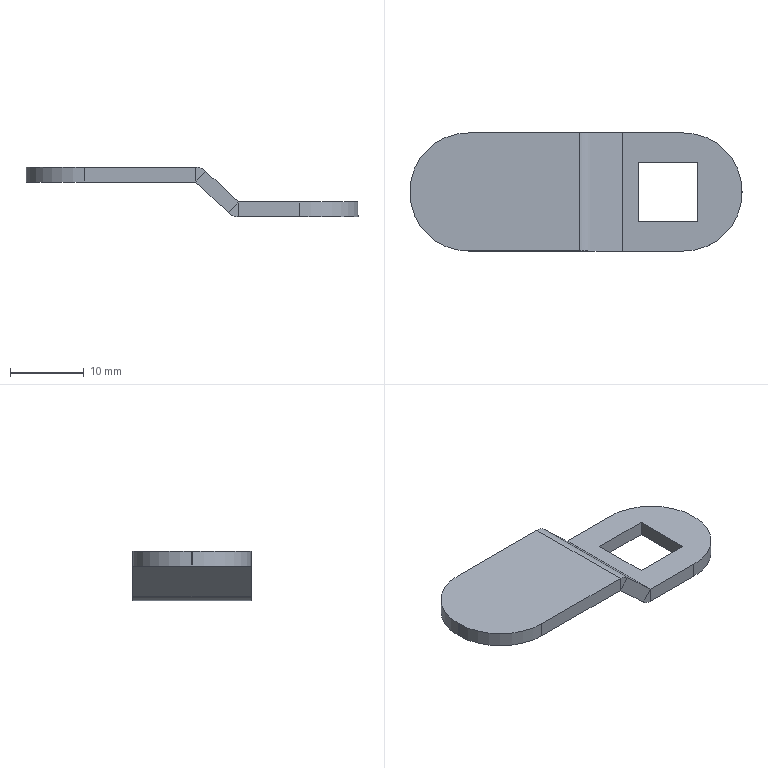Component | SolidWorks | LeftDoorPanelAssembly-1_LockPlate-1 | 1 solid | 30 faces | box 45 x 16 x 6.7 mm | volume 1262 mm3 | plane 22 | cylinder 8 | commonest cylinder face diameters 15.8 x4 0.08 x2 4.08 x2
STEP:
#1=COLOUR_RGB('',0.7922,0.8196,0.9333);
#2=FILL_AREA_STYLE_COLOUR('',#1);
#3=FILL_AREA_STYLE('',(#2));
#4=SURFACE_STYLE_FILL_AREA(#3);
#5=SURFACE_SIDE_STYLE('',(#4));
#6=SURFACE_STYLE_USAGE(.BOTH.,#5);
#7=PRESENTATION_STYLE_ASSIGNMENT((#6));
#8=CARTESIAN_POINT('',(-0.2747,0.2182,-2.108));
#9=VERTEX_POINT('',#8);
#10=CARTESIAN_POINT('',(-0.2208,0.2182,-2.051));
#11=VERTEX_POINT('',#10);
#12=CARTESIAN_POINT('',(-0.2747,0.2182,-2.108));
#13=DIRECTION('',(0.6849,0.,0.7286));
#14=VECTOR('',#13,39.37);
#15=LINE('',#12,#14);
#16=EDGE_CURVE('',#9,#11,#15,.T.);
#17=ORIENTED_EDGE('',*,*,#16,.F.);
#18=CARTESIAN_POINT('',(-0.2197,0.2182,-2.13));
#19=VERTEX_POINT('',#18);
#20=CARTESIAN_POINT('',(-0.2197,0.2182,-2.05));
#21=DIRECTION('',(-0.,1.,-0.));
#22=DIRECTION('',(-1.,-0.,-0.));
#23=AXIS2_PLACEMENT_3D('',#20,#21,#22);
#24=CIRCLE('',#23,0.08031);
#25=EDGE_CURVE('',#19,#9,#24,.T.);
#26=ORIENTED_EDGE('',*,*,#25,.F.);
#27=CARTESIAN_POINT('',(-0.2197,0.2182,-2.051));
#28=VERTEX_POINT('',#27);
#29=CARTESIAN_POINT('',(-0.2197,0.2182,-2.051));
#30=DIRECTION('',(0.,-0.,-1.));
#31=VECTOR('',#30,39.37);
#32=LINE('',#29,#31);
#33=EDGE_CURVE('',#28,#19,#32,.T.);
#34=ORIENTED_EDGE('',*,*,#33,.F.);
#35=CARTESIAN_POINT('',(-0.2197,0.2182,-2.05));
#36=DIRECTION('',(-0.,1.,-0.));
#37=DIRECTION('',(-1.,0.,0.));
#38=AXIS2_PLACEMENT_3D('',#35,#36,#37);
#39=CIRCLE('',#38,0.001575);
#40=EDGE_CURVE('',#28,#11,#39,.T.);
#41=ORIENTED_EDGE('',*,*,#40,.T.);
#42=EDGE_LOOP('',(#17,#26,#34,#41));
#43=FACE_OUTER_BOUND('',#42,.T.);
#44=CARTESIAN_POINT('',(-0.2747,0.2182,-2.108));
#45=DIRECTION('',(0.,-1.,0.));
#46=DIRECTION('',(-1.,-0.,-0.));
#47=AXIS2_PLACEMENT_3D('',#44,#45,#46);
#48=PLANE('',#47);
#49=ADVANCED_FACE('',(#43),#48,.T.);
#50=CARTESIAN_POINT('',(-0.4479,0.2182,-1.945));
#51=VERTEX_POINT('',#50);
#52=CARTESIAN_POINT('',(-0.2515,0.2182,-2.13));
#53=DIRECTION('',(-0.7286,0.,0.6849));
#54=VECTOR('',#53,39.37);
#55=LINE('',#52,#54);
#56=EDGE_CURVE('',#9,#51,#55,.T.);
#57=ORIENTED_EDGE('',*,*,#56,.F.);
#58=ORIENTED_EDGE('',*,*,#16,.T.);
#59=CARTESIAN_POINT('',(-0.394,0.2182,-1.888));
#60=VERTEX_POINT('',#59);
#61=CARTESIAN_POINT('',(-0.1976,0.2182,-2.073));
#62=DIRECTION('',(-0.7286,0.,0.6849));
#63=VECTOR('',#62,39.37);
#64=LINE('',#61,#63);
#65=EDGE_CURVE('',#11,#60,#64,.T.);
#66=ORIENTED_EDGE('',*,*,#65,.T.);
#67=CARTESIAN_POINT('',(-0.394,0.2182,-1.888));
#68=DIRECTION('',(-0.6849,-0.,-0.7286));
#69=VECTOR('',#68,39.37);
#70=LINE('',#67,#69);
#71=EDGE_CURVE('',#60,#51,#70,.T.);
#72=ORIENTED_EDGE('',*,*,#71,.T.);
#73=EDGE_LOOP('',(#57,#58,#66,#72));
#74=FACE_OUTER_BOUND('',#73,.T.);
#75=CARTESIAN_POINT('',(-0.2197,0.2182,-2.051));
#76=DIRECTION('',(0.,-1.,0.));
#77=DIRECTION('',(-1.,-0.,-0.));
#78=AXIS2_PLACEMENT_3D('',#75,#76,#77);
#79=PLANE('',#78);
#80=ADVANCED_FACE('',(#74),#79,.T.);
#81=CARTESIAN_POINT('',(-0.2197,0.8481,-2.13));
#82=VERTEX_POINT('',#81);
#83=CARTESIAN_POINT('',(-0.2197,0.8481,-2.051));
#84=VERTEX_POINT('',#83);
#85=CARTESIAN_POINT('',(-0.2197,0.8481,-2.13));
#86=DIRECTION('',(-0.,0.,1.));
#87=VECTOR('',#86,39.37);
#88=LINE('',#85,#87);
#89=EDGE_CURVE('',#82,#84,#88,.T.);
#90=ORIENTED_EDGE('',*,*,#89,.F.);
#91=CARTESIAN_POINT('',(-0.2747,0.8481,-2.108));
#92=VERTEX_POINT('',#91);
#93=CARTESIAN_POINT('',(-0.2197,0.8481,-2.05));
#94=DIRECTION('',(-0.,1.,-0.));
#95=DIRECTION('',(-1.,-0.,-0.));
#96=AXIS2_PLACEMENT_3D('',#93,#94,#95);
#97=CIRCLE('',#96,0.08031);
#98=EDGE_CURVE('',#82,#92,#97,.T.);
#99=ORIENTED_EDGE('',*,*,#98,.T.);
#100=CARTESIAN_POINT('',(-0.2208,0.8481,-2.051));
#101=VERTEX_POINT('',#100);
#102=CARTESIAN_POINT('',(-0.2208,0.8481,-2.051));
#103=DIRECTION('',(-0.6849,-0.,-0.7286));
#104=VECTOR('',#103,39.37);
#105=LINE('',#102,#104);
#106=EDGE_CURVE('',#101,#92,#105,.T.);
#107=ORIENTED_EDGE('',*,*,#106,.F.);
#108=CARTESIAN_POINT('',(-0.2197,0.8481,-2.05));
#109=DIRECTION('',(-0.,1.,-0.));
#110=DIRECTION('',(-1.,0.,0.));
#111=AXIS2_PLACEMENT_3D('',#108,#109,#110);
#112=CIRCLE('',#111,0.001575);
#113=EDGE_CURVE('',#84,#101,#112,.T.);
#114=ORIENTED_EDGE('',*,*,#113,.F.);
#115=EDGE_LOOP('',(#90,#99,#107,#114));
#116=FACE_OUTER_BOUND('',#115,.T.);
#117=CARTESIAN_POINT('',(-0.2197,0.8481,-2.13));
#118=DIRECTION('',(-0.,1.,-0.));
#119=DIRECTION('',(1.,0.,0.));
#120=AXIS2_PLACEMENT_3D('',#117,#118,#119);
#121=PLANE('',#120);
#122=ADVANCED_FACE('',(#116),#121,.T.);
#123=CARTESIAN_POINT('',(0.1068,0.8481,-2.051));
#124=VERTEX_POINT('',#123);
#125=CARTESIAN_POINT('',(0.4178,0.8481,-2.051));
#126=DIRECTION('',(-1.,-0.,-0.));
#127=VECTOR('',#126,39.37);
#128=LINE('',#125,#127);
#129=EDGE_CURVE('',#124,#84,#128,.T.);
#130=ORIENTED_EDGE('',*,*,#129,.F.);
#131=CARTESIAN_POINT('',(0.1068,0.8481,-2.13));
#132=VERTEX_POINT('',#131);
#133=CARTESIAN_POINT('',(0.1068,0.8481,-2.051));
#134=DIRECTION('',(0.,-0.,-1.));
#135=VECTOR('',#134,39.37);
#136=LINE('',#133,#135);
#137=EDGE_CURVE('',#124,#132,#136,.T.);
#138=ORIENTED_EDGE('',*,*,#137,.T.);
#139=CARTESIAN_POINT('',(0.4178,0.8481,-2.13));
#140=DIRECTION('',(-1.,-0.,-0.));
#141=VECTOR('',#140,39.37);
#142=LINE('',#139,#141);
#143=EDGE_CURVE('',#132,#82,#142,.T.);
#144=ORIENTED_EDGE('',*,*,#143,.T.);
#145=ORIENTED_EDGE('',*,*,#89,.T.);
#146=EDGE_LOOP('',(#130,#138,#144,#145));
#147=FACE_OUTER_BOUND('',#146,.T.);
#148=CARTESIAN_POINT('',(-0.2208,0.8481,-2.051));
#149=DIRECTION('',(-0.,1.,-0.));
#150=DIRECTION('',(1.,0.,0.));
#151=AXIS2_PLACEMENT_3D('',#148,#149,#150);
#152=PLANE('',#151);
#153=ADVANCED_FACE('',(#147),#152,.T.);
#154=CARTESIAN_POINT('',(-0.449,0.2182,-1.945));
#155=VERTEX_POINT('',#154);
#156=CARTESIAN_POINT('',(-0.449,0.2182,-1.866));
#157=VERTEX_POINT('',#156);
#158=CARTESIAN_POINT('',(-0.449,0.2182,-1.945));
#159=DIRECTION('',(-0.,0.,1.));
#160=VECTOR('',#159,39.37);
#161=LINE('',#158,#160);
#162=EDGE_CURVE('',#155,#157,#161,.T.);
#163=ORIENTED_EDGE('',*,*,#162,.F.);
#164=CARTESIAN_POINT('',(-0.449,0.2182,-1.946));
#165=DIRECTION('',(0.,-1.,0.));
#166=DIRECTION('',(1.,0.,0.));
#167=AXIS2_PLACEMENT_3D('',#164,#165,#166);
#168=CIRCLE('',#167,0.001575);
#169=EDGE_CURVE('',#51,#155,#168,.T.);
#170=ORIENTED_EDGE('',*,*,#169,.F.);
#171=ORIENTED_EDGE('',*,*,#71,.F.);
#172=CARTESIAN_POINT('',(-0.449,0.2182,-1.946));
#173=DIRECTION('',(0.,-1.,0.));
#174=DIRECTION('',(-1.,-0.,-0.));
#175=AXIS2_PLACEMENT_3D('',#172,#173,#174);
#176=CIRCLE('',#175,0.08031);
#177=EDGE_CURVE('',#60,#157,#176,.T.);
#178=ORIENTED_EDGE('',*,*,#177,.T.);
#179=EDGE_LOOP('',(#163,#170,#171,#178));
#180=FACE_OUTER_BOUND('',#179,.T.);
#181=CARTESIAN_POINT('',(-0.449,0.2182,-1.945));
#182=DIRECTION('',(0.,-1.,0.));
#183=DIRECTION('',(-1.,-0.,-0.));
#184=AXIS2_PLACEMENT_3D('',#181,#182,#183);
#185=PLANE('',#184);
#186=ADVANCED_FACE('',(#180),#185,.T.);
#187=CARTESIAN_POINT('',(-1.043,0.2182,-1.866));
#188=VERTEX_POINT('',#187);
#189=CARTESIAN_POINT('',(-0.4484,0.2182,-1.866));
#190=DIRECTION('',(-1.,-0.,-0.));
#191=VECTOR('',#190,39.37);
#192=LINE('',#189,#191);
#193=EDGE_CURVE('',#157,#188,#192,.T.);
#194=ORIENTED_EDGE('',*,*,#193,.T.);
#195=CARTESIAN_POINT('',(-1.043,0.2182,-1.945));
#196=VERTEX_POINT('',#195);
#197=CARTESIAN_POINT('',(-1.043,0.2182,-1.888));
#198=DIRECTION('',(0.,-0.,-1.));
#199=VECTOR('',#198,39.37);
#200=LINE('',#197,#199);
#201=EDGE_CURVE('',#188,#196,#200,.T.);
#202=ORIENTED_EDGE('',*,*,#201,.T.);
#203=CARTESIAN_POINT('',(-0.4484,0.2182,-1.945));
#204=DIRECTION('',(-1.,-0.,-0.));
#205=VECTOR('',#204,39.37);
#206=LINE('',#203,#205);
#207=EDGE_CURVE('',#155,#196,#206,.T.);
#208=ORIENTED_EDGE('',*,*,#207,.F.);
#209=ORIENTED_EDGE('',*,*,#162,.T.);
#210=EDGE_LOOP('',(#194,#202,#208,#209));
#211=FACE_OUTER_BOUND('',#210,.T.);
#212=CARTESIAN_POINT('',(-0.394,0.2182,-1.888));
#213=DIRECTION('',(0.,-1.,0.));
#214=DIRECTION('',(-1.,-0.,-0.));
#215=AXIS2_PLACEMENT_3D('',#212,#213,#214);
#216=PLANE('',#215);
#217=ADVANCED_FACE('',(#211),#216,.T.);
#218=CARTESIAN_POINT('',(-0.4479,0.8481,-1.945));
#219=VERTEX_POINT('',#218);
#220=CARTESIAN_POINT('',(-0.394,0.8481,-1.888));
#221=VERTEX_POINT('',#220);
#222=CARTESIAN_POINT('',(-0.4479,0.8481,-1.945));
#223=DIRECTION('',(0.6849,0.,0.7286));
#224=VECTOR('',#223,39.37);
#225=LINE('',#222,#224);
#226=EDGE_CURVE('',#219,#221,#225,.T.);
#227=ORIENTED_EDGE('',*,*,#226,.F.);
#228=CARTESIAN_POINT('',(-0.449,0.8481,-1.945));
#229=VERTEX_POINT('',#228);
#230=CARTESIAN_POINT('',(-0.449,0.8481,-1.946));
#231=DIRECTION('',(0.,-1.,0.));
#232=DIRECTION('',(1.,0.,0.));
#233=AXIS2_PLACEMENT_3D('',#230,#231,#232);
#234=CIRCLE('',#233,0.001575);
#235=EDGE_CURVE('',#219,#229,#234,.T.);
#236=ORIENTED_EDGE('',*,*,#235,.T.);
#237=CARTESIAN_POINT('',(-0.449,0.8481,-1.866));
#238=VERTEX_POINT('',#237);
#239=CARTESIAN_POINT('',(-0.449,0.8481,-1.866));
#240=DIRECTION('',(0.,-0.,-1.));
#241=VECTOR('',#240,39.37);
#242=LINE('',#239,#241);
#243=EDGE_CURVE('',#238,#229,#242,.T.);
#244=ORIENTED_EDGE('',*,*,#243,.F.);
#245=CARTESIAN_POINT('',(-0.449,0.8481,-1.946));
#246=DIRECTION('',(0.,-1.,0.));
#247=DIRECTION('',(-1.,-0.,-0.));
#248=AXIS2_PLACEMENT_3D('',#245,#246,#247);
#249=CIRCLE('',#248,0.08031);
#250=EDGE_CURVE('',#221,#238,#249,.T.);
#251=ORIENTED_EDGE('',*,*,#250,.F.);
#252=EDGE_LOOP('',(#227,#236,#244,#251));
#253=FACE_OUTER_BOUND('',#252,.T.);
#254=CARTESIAN_POINT('',(-0.4479,0.8481,-1.945));
#255=DIRECTION('',(-0.,1.,-0.));
#256=DIRECTION('',(1.,0.,0.));
#257=AXIS2_PLACEMENT_3D('',#254,#255,#256);
#258=PLANE('',#257);
#259=ADVANCED_FACE('',(#253),#258,.T.);
#260=CARTESIAN_POINT('',(-0.2515,0.8481,-2.13));
#261=DIRECTION('',(-0.7286,0.,0.6849));
#262=VECTOR('',#261,39.37);
#263=LINE('',#260,#262);
#264=EDGE_CURVE('',#92,#219,#263,.T.);
#265=ORIENTED_EDGE('',*,*,#264,.T.);
#266=ORIENTED_EDGE('',*,*,#226,.T.);
#267=CARTESIAN_POINT('',(-0.1976,0.8481,-2.073));
#268=DIRECTION('',(-0.7286,0.,0.6849));
#269=VECTOR('',#268,39.37);
#270=LINE('',#267,#269);
#271=EDGE_CURVE('',#101,#221,#270,.T.);
#272=ORIENTED_EDGE('',*,*,#271,.F.);
#273=ORIENTED_EDGE('',*,*,#106,.T.);
#274=EDGE_LOOP('',(#265,#266,#272,#273));
#275=FACE_OUTER_BOUND('',#274,.T.);
#276=CARTESIAN_POINT('',(-0.449,0.8481,-1.866));
#277=DIRECTION('',(-0.,1.,-0.));
#278=DIRECTION('',(1.,0.,0.));
#279=AXIS2_PLACEMENT_3D('',#276,#277,#278);
#280=PLANE('',#279);
#281=ADVANCED_FACE('',(#275),#280,.T.);
#282=CARTESIAN_POINT('',(-1.354,0.5292,-1.866));
#283=VERTEX_POINT('',#282);
#284=CARTESIAN_POINT('',(-1.354,0.5371,-1.866));
#285=VERTEX_POINT('',#284);
#286=CARTESIAN_POINT('',(-1.354,0.2182,-1.866));
#287=DIRECTION('',(-0.,1.,-0.));
#288=VECTOR('',#287,39.37);
#289=LINE('',#286,#288);
#290=EDGE_CURVE('',#283,#285,#289,.T.);
#291=ORIENTED_EDGE('',*,*,#290,.F.);
#292=CARTESIAN_POINT('',(-1.043,0.5292,-1.866));
#293=DIRECTION('',(-0.,0.,1.));
#294=DIRECTION('',(0.,-1.,0.));
#295=AXIS2_PLACEMENT_3D('',#292,#293,#294);
#296=CIRCLE('',#295,0.311);
#297=EDGE_CURVE('',#283,#188,#296,.T.);
#298=ORIENTED_EDGE('',*,*,#297,.T.);
#299=ORIENTED_EDGE('',*,*,#193,.F.);
#300=CARTESIAN_POINT('',(-0.449,0.2182,-1.866));
#301=DIRECTION('',(-0.,1.,-0.));
#302=VECTOR('',#301,39.37);
#303=LINE('',#300,#302);
#304=EDGE_CURVE('',#157,#238,#303,.T.);
#305=ORIENTED_EDGE('',*,*,#304,.T.);
#306=CARTESIAN_POINT('',(-1.043,0.8481,-1.866));
#307=VERTEX_POINT('',#306);
#308=CARTESIAN_POINT('',(-0.4484,0.8481,-1.866));
#309=DIRECTION('',(-1.,-0.,-0.));
#310=VECTOR('',#309,39.37);
#311=LINE('',#308,#310);
#312=EDGE_CURVE('',#238,#307,#311,.T.);
#313=ORIENTED_EDGE('',*,*,#312,.T.);
#314=CARTESIAN_POINT('',(-1.043,0.5371,-1.866));
#315=DIRECTION('',(-0.,0.,1.));
#316=DIRECTION('',(0.,-1.,0.));
#317=AXIS2_PLACEMENT_3D('',#314,#315,#316);
#318=CIRCLE('',#317,0.311);
#319=EDGE_CURVE('',#307,#285,#318,.T.);
#320=ORIENTED_EDGE('',*,*,#319,.T.);
#321=EDGE_LOOP('',(#291,#298,#299,#305,#313,#320));
#322=FACE_OUTER_BOUND('',#321,.T.);
#323=CARTESIAN_POINT('',(-0.4484,0.2182,-1.866));
#324=DIRECTION('',(0.,-0.,-1.));
#325=DIRECTION('',(0.,-1.,0.));
#326=AXIS2_PLACEMENT_3D('',#323,#324,#325);
#327=PLANE('',#326);
#328=ADVANCED_FACE('',(#322),#327,.F.);
#329=CARTESIAN_POINT('',(-1.354,0.5292,-1.945));
#330=VERTEX_POINT('',#329);
#331=CARTESIAN_POINT('',(-1.354,0.5371,-1.945));
#332=VERTEX_POINT('',#331);
#333=CARTESIAN_POINT('',(-1.354,0.2182,-1.945));
#334=DIRECTION('',(-0.,1.,-0.));
#335=VECTOR('',#334,39.37);
#336=LINE('',#333,#335);
#337=EDGE_CURVE('',#330,#332,#336,.T.);
#338=ORIENTED_EDGE('',*,*,#337,.F.);
#339=CARTESIAN_POINT('',(-1.354,0.5292,-1.945));
#340=DIRECTION('',(-0.,0.,1.));
#341=VECTOR('',#340,39.37);
#342=LINE('',#339,#341);
#343=EDGE_CURVE('',#330,#283,#342,.T.);
#344=ORIENTED_EDGE('',*,*,#343,.T.);
#345=ORIENTED_EDGE('',*,*,#290,.T.);
#346=CARTESIAN_POINT('',(-1.354,0.5371,-1.945));
#347=DIRECTION('',(0.,-0.,-1.));
#348=VECTOR('',#347,39.37);
#349=LINE('',#346,#348);
#350=EDGE_CURVE('',#285,#332,#349,.T.);
#351=ORIENTED_EDGE('',*,*,#350,.T.);
#352=EDGE_LOOP('',(#338,#344,#345,#351));
#353=FACE_OUTER_BOUND('',#352,.T.);
#354=CARTESIAN_POINT('',(-1.354,0.2182,-1.945));
#355=DIRECTION('',(-1.,-0.,-0.));
#356=DIRECTION('',(-0.,1.,-0.));
#357=AXIS2_PLACEMENT_3D('',#354,#355,#356);
#358=PLANE('',#357);
#359=ADVANCED_FACE('',(#353),#358,.T.);
#360=ORIENTED_EDGE('',*,*,#207,.T.);
#361=CARTESIAN_POINT('',(-1.043,0.5292,-1.945));
#362=DIRECTION('',(0.,-0.,-1.));
#363=DIRECTION('',(0.,-1.,0.));
#364=AXIS2_PLACEMENT_3D('',#361,#362,#363);
#365=CIRCLE('',#364,0.311);
#366=EDGE_CURVE('',#196,#330,#365,.T.);
#367=ORIENTED_EDGE('',*,*,#366,.T.);
#368=ORIENTED_EDGE('',*,*,#337,.T.);
#369=CARTESIAN_POINT('',(-1.043,0.8481,-1.945));
#370=VERTEX_POINT('',#369);
#371=CARTESIAN_POINT('',(-1.043,0.5371,-1.945));
#372=DIRECTION('',(0.,-0.,-1.));
#373=DIRECTION('',(0.,-1.,0.));
#374=AXIS2_PLACEMENT_3D('',#371,#372,#373);
#375=CIRCLE('',#374,0.311);
#376=EDGE_CURVE('',#332,#370,#375,.T.);
#377=ORIENTED_EDGE('',*,*,#376,.T.);
#378=CARTESIAN_POINT('',(-0.4484,0.8481,-1.945));
#379=DIRECTION('',(-1.,-0.,-0.));
#380=VECTOR('',#379,39.37);
#381=LINE('',#378,#380);
#382=EDGE_CURVE('',#229,#370,#381,.T.);
#383=ORIENTED_EDGE('',*,*,#382,.F.);
#384=CARTESIAN_POINT('',(-0.449,0.2182,-1.945));
#385=DIRECTION('',(-0.,1.,-0.));
#386=VECTOR('',#385,39.37);
#387=LINE('',#384,#386);
#388=EDGE_CURVE('',#155,#229,#387,.T.);
#389=ORIENTED_EDGE('',*,*,#388,.F.);
#390=EDGE_LOOP('',(#360,#367,#368,#377,#383,#389));
#391=FACE_OUTER_BOUND('',#390,.T.);
#392=CARTESIAN_POINT('',(-0.4484,0.2182,-1.945));
#393=DIRECTION('',(0.,-0.,-1.));
#394=DIRECTION('',(0.,-1.,0.));
#395=AXIS2_PLACEMENT_3D('',#392,#393,#394);
#396=PLANE('',#395);
#397=ADVANCED_FACE('',(#391),#396,.T.);
#398=ORIENTED_EDGE('',*,*,#235,.F.);
#399=CARTESIAN_POINT('',(-0.4479,0.2182,-1.945));
#400=DIRECTION('',(-0.,1.,-0.));
#401=VECTOR('',#400,39.37);
#402=LINE('',#399,#401);
#403=EDGE_CURVE('',#51,#219,#402,.T.);
#404=ORIENTED_EDGE('',*,*,#403,.F.);
#405=ORIENTED_EDGE('',*,*,#169,.T.);
#406=ORIENTED_EDGE('',*,*,#388,.T.);
#407=EDGE_LOOP('',(#398,#404,#405,#406));
#408=FACE_OUTER_BOUND('',#407,.T.);
#409=CARTESIAN_POINT('',(-0.449,0.2182,-1.946));
#410=DIRECTION('',(-0.,1.,-0.));
#411=DIRECTION('',(1.,0.,0.));
#412=AXIS2_PLACEMENT_3D('',#409,#410,#411);
#413=CYLINDRICAL_SURFACE('',#412,0.001575);
#414=ADVANCED_FACE('',(#408),#413,.F.);
#415=ORIENTED_EDGE('',*,*,#264,.F.);
#416=CARTESIAN_POINT('',(-0.2747,0.2182,-2.108));
#417=DIRECTION('',(-0.,1.,-0.));
#418=VECTOR('',#417,39.37);
#419=LINE('',#416,#418);
#420=EDGE_CURVE('',#9,#92,#419,.T.);
#421=ORIENTED_EDGE('',*,*,#420,.F.);
#422=ORIENTED_EDGE('',*,*,#56,.T.);
#423=ORIENTED_EDGE('',*,*,#403,.T.);
#424=EDGE_LOOP('',(#415,#421,#422,#423));
#425=FACE_OUTER_BOUND('',#424,.T.);
#426=CARTESIAN_POINT('',(-0.2515,0.2182,-2.13));
#427=DIRECTION('',(-0.6849,-0.,-0.7286));
#428=DIRECTION('',(0.7286,-0.,-0.6849));
#429=AXIS2_PLACEMENT_3D('',#426,#427,#428);
#430=PLANE('',#429);
#431=ADVANCED_FACE('',(#425),#430,.T.);
#432=ORIENTED_EDGE('',*,*,#98,.F.);
#433=CARTESIAN_POINT('',(-0.2197,0.2182,-2.13));
#434=DIRECTION('',(-0.,1.,-0.));
#435=VECTOR('',#434,39.37);
#436=LINE('',#433,#435);
#437=EDGE_CURVE('',#19,#82,#436,.T.);
#438=ORIENTED_EDGE('',*,*,#437,.F.);
#439=ORIENTED_EDGE('',*,*,#25,.T.);
#440=ORIENTED_EDGE('',*,*,#420,.T.);
#441=EDGE_LOOP('',(#432,#438,#439,#440));
#442=FACE_OUTER_BOUND('',#441,.T.);
#443=CARTESIAN_POINT('',(-0.2197,0.2182,-2.05));
#444=DIRECTION('',(-0.,1.,-0.));
#445=DIRECTION('',(1.,0.,0.));
#446=AXIS2_PLACEMENT_3D('',#443,#444,#445);
#447=CYLINDRICAL_SURFACE('',#446,0.08031);
#448=ADVANCED_FACE('',(#442),#447,.T.);
#449=CARTESIAN_POINT('',(-0.1334,0.3757,-2.13));
#450=VERTEX_POINT('',#449);
#451=CARTESIAN_POINT('',(-0.1334,0.6906,-2.13));
#452=VERTEX_POINT('',#451);
#453=CARTESIAN_POINT('',(-0.1334,0.6906,-2.13));
#454=DIRECTION('',(-0.,1.,-0.));
#455=VECTOR('',#454,39.37);
#456=LINE('',#453,#455);
#457=EDGE_CURVE('',#450,#452,#456,.T.);
#458=ORIENTED_EDGE('',*,*,#457,.F.);
#459=CARTESIAN_POINT('',(0.1816,0.3757,-2.13));
#460=VERTEX_POINT('',#459);
#461=CARTESIAN_POINT('',(0.1816,0.3757,-2.13));
#462=DIRECTION('',(-1.,-0.,-0.));
#463=VECTOR('',#462,39.37);
#464=LINE('',#461,#463);
#465=EDGE_CURVE('',#460,#450,#464,.T.);
#466=ORIENTED_EDGE('',*,*,#465,.F.);
#467=CARTESIAN_POINT('',(0.1816,0.6906,-2.13));
#468=VERTEX_POINT('',#467);
#469=CARTESIAN_POINT('',(0.1816,0.6906,-2.13));
#470=DIRECTION('',(0.,-1.,0.));
#471=VECTOR('',#470,39.37);
#472=LINE('',#469,#471);
#473=EDGE_CURVE('',#468,#460,#472,.T.);
#474=ORIENTED_EDGE('',*,*,#473,.F.);
#475=CARTESIAN_POINT('',(0.1816,0.6906,-2.13));
#476=DIRECTION('',(1.,0.,0.));
#477=VECTOR('',#476,39.37);
#478=LINE('',#475,#477);
#479=EDGE_CURVE('',#452,#468,#478,.T.);
#480=ORIENTED_EDGE('',*,*,#479,.F.);
#481=EDGE_LOOP('',(#458,#466,#474,#480));
#482=FACE_BOUND('',#481,.T.);
#483=CARTESIAN_POINT('',(0.4178,0.5292,-2.13));
#484=VERTEX_POINT('',#483);
#485=CARTESIAN_POINT('',(0.4178,0.5371,-2.13));
#486=VERTEX_POINT('',#485);
#487=CARTESIAN_POINT('',(0.4178,0.2182,-2.13));
#488=DIRECTION('',(-0.,1.,-0.));
#489=VECTOR('',#488,39.37);
#490=LINE('',#487,#489);
#491=EDGE_CURVE('',#484,#486,#490,.T.);
#492=ORIENTED_EDGE('',*,*,#491,.F.);
#493=CARTESIAN_POINT('',(0.1068,0.2182,-2.13));
#494=VERTEX_POINT('',#493);
#495=CARTESIAN_POINT('',(0.1068,0.5292,-2.13));
#496=DIRECTION('',(0.,-0.,-1.));
#497=DIRECTION('',(0.,-1.,0.));
#498=AXIS2_PLACEMENT_3D('',#495,#496,#497);
#499=CIRCLE('',#498,0.311);
#500=EDGE_CURVE('',#484,#494,#499,.T.);
#501=ORIENTED_EDGE('',*,*,#500,.T.);
#502=CARTESIAN_POINT('',(0.4178,0.2182,-2.13));
#503=DIRECTION('',(-1.,-0.,-0.));
#504=VECTOR('',#503,39.37);
#505=LINE('',#502,#504);
#506=EDGE_CURVE('',#494,#19,#505,.T.);
#507=ORIENTED_EDGE('',*,*,#506,.T.);
#508=ORIENTED_EDGE('',*,*,#437,.T.);
#509=ORIENTED_EDGE('',*,*,#143,.F.);
#510=CARTESIAN_POINT('',(0.1068,0.5371,-2.13));
#511=DIRECTION('',(0.,-0.,-1.));
#512=DIRECTION('',(0.,-1.,0.));
#513=AXIS2_PLACEMENT_3D('',#510,#511,#512);
#514=CIRCLE('',#513,0.311);
#515=EDGE_CURVE('',#132,#486,#514,.T.);
#516=ORIENTED_EDGE('',*,*,#515,.T.);
#517=EDGE_LOOP('',(#492,#501,#507,#508,#509,#516));
#518=FACE_OUTER_BOUND('',#517,.T.);
#519=CARTESIAN_POINT('',(0.4178,0.2182,-2.13));
#520=DIRECTION('',(0.,-0.,-1.));
#521=DIRECTION('',(0.,-1.,0.));
#522=AXIS2_PLACEMENT_3D('',#519,#520,#521);
#523=PLANE('',#522);
#524=ADVANCED_FACE('',(#482,#518),#523,.T.);
#525=CARTESIAN_POINT('',(0.4178,0.5292,-2.051));
#526=VERTEX_POINT('',#525);
#527=CARTESIAN_POINT('',(0.4178,0.5371,-2.051));
#528=VERTEX_POINT('',#527);
#529=CARTESIAN_POINT('',(0.4178,0.2182,-2.051));
#530=DIRECTION('',(-0.,1.,-0.));
#531=VECTOR('',#530,39.37);
#532=LINE('',#529,#531);
#533=EDGE_CURVE('',#526,#528,#532,.T.);
#534=ORIENTED_EDGE('',*,*,#533,.F.);
#535=CARTESIAN_POINT('',(0.4178,0.5292,-2.13));
#536=DIRECTION('',(0.,-0.,-1.));
#537=VECTOR('',#536,39.37);
#538=LINE('',#535,#537);
#539=EDGE_CURVE('',#526,#484,#538,.T.);
#540=ORIENTED_EDGE('',*,*,#539,.T.);
#541=ORIENTED_EDGE('',*,*,#491,.T.);
#542=CARTESIAN_POINT('',(0.4178,0.5371,-2.051));
#543=DIRECTION('',(-0.,0.,1.));
#544=VECTOR('',#543,39.37);
#545=LINE('',#542,#544);
#546=EDGE_CURVE('',#486,#528,#545,.T.);
#547=ORIENTED_EDGE('',*,*,#546,.T.);
#548=EDGE_LOOP('',(#534,#540,#541,#547));
#549=FACE_OUTER_BOUND('',#548,.T.);
#550=CARTESIAN_POINT('',(0.4178,0.2182,-2.051));
#551=DIRECTION('',(1.,0.,0.));
#552=DIRECTION('',(0.,-1.,0.));
#553=AXIS2_PLACEMENT_3D('',#550,#551,#552);
#554=PLANE('',#553);
#555=ADVANCED_FACE('',(#549),#554,.T.);
#556=CARTESIAN_POINT('',(0.1816,0.3757,-2.051));
#557=VERTEX_POINT('',#556);
#558=CARTESIAN_POINT('',(-0.1334,0.3757,-2.051));
#559=VERTEX_POINT('',#558);
#560=CARTESIAN_POINT('',(0.4178,0.3757,-2.051));
#561=DIRECTION('',(-1.,-0.,-0.));
#562=VECTOR('',#561,39.37);
#563=LINE('',#560,#562);
#564=EDGE_CURVE('',#557,#559,#563,.T.);
#565=ORIENTED_EDGE('',*,*,#564,.T.);
#566=CARTESIAN_POINT('',(-0.1334,0.6906,-2.051));
#567=VERTEX_POINT('',#566);
#568=CARTESIAN_POINT('',(-0.1334,0.2182,-2.051));
#569=DIRECTION('',(-0.,1.,-0.));
#570=VECTOR('',#569,39.37);
#571=LINE('',#568,#570);
#572=EDGE_CURVE('',#559,#567,#571,.T.);
#573=ORIENTED_EDGE('',*,*,#572,.T.);
#574=CARTESIAN_POINT('',(0.1816,0.6906,-2.051));
#575=VERTEX_POINT('',#574);
#576=CARTESIAN_POINT('',(0.4178,0.6906,-2.051));
#577=DIRECTION('',(1.,0.,0.));
#578=VECTOR('',#577,39.37);
#579=LINE('',#576,#578);
#580=EDGE_CURVE('',#567,#575,#579,.T.);
#581=ORIENTED_EDGE('',*,*,#580,.T.);
#582=CARTESIAN_POINT('',(0.1816,0.2182,-2.051));
#583=DIRECTION('',(0.,-1.,0.));
#584=VECTOR('',#583,39.37);
#585=LINE('',#582,#584);
#586=EDGE_CURVE('',#575,#557,#585,.T.);
#587=ORIENTED_EDGE('',*,*,#586,.T.);
#588=EDGE_LOOP('',(#565,#573,#581,#587));
#589=FACE_BOUND('',#588,.T.);
#590=CARTESIAN_POINT('',(0.1068,0.2182,-2.051));
#591=VERTEX_POINT('',#590);
#592=CARTESIAN_POINT('',(0.4178,0.2182,-2.051));
#593=DIRECTION('',(-1.,-0.,-0.));
#594=VECTOR('',#593,39.37);
#595=LINE('',#592,#594);
#596=EDGE_CURVE('',#591,#28,#595,.T.);
#597=ORIENTED_EDGE('',*,*,#596,.F.);
#598=CARTESIAN_POINT('',(0.1068,0.5292,-2.051));
#599=DIRECTION('',(-0.,0.,1.));
#600=DIRECTION('',(0.,-1.,0.));
#601=AXIS2_PLACEMENT_3D('',#598,#599,#600);
#602=CIRCLE('',#601,0.311);
#603=EDGE_CURVE('',#591,#526,#602,.T.);
#604=ORIENTED_EDGE('',*,*,#603,.T.);
#605=ORIENTED_EDGE('',*,*,#533,.T.);
#606=CARTESIAN_POINT('',(0.1068,0.5371,-2.051));
#607=DIRECTION('',(-0.,0.,1.));
#608=DIRECTION('',(0.,-1.,0.));
#609=AXIS2_PLACEMENT_3D('',#606,#607,#608);
#610=CIRCLE('',#609,0.311);
#611=EDGE_CURVE('',#528,#124,#610,.T.);
#612=ORIENTED_EDGE('',*,*,#611,.T.);
#613=ORIENTED_EDGE('',*,*,#129,.T.);
#614=CARTESIAN_POINT('',(-0.2197,0.2182,-2.051));
#615=DIRECTION('',(-0.,1.,-0.));
#616=VECTOR('',#615,39.37);
#617=LINE('',#614,#616);
#618=EDGE_CURVE('',#28,#84,#617,.T.);
#619=ORIENTED_EDGE('',*,*,#618,.F.);
#620=EDGE_LOOP('',(#597,#604,#605,#612,#613,#619));
#621=FACE_OUTER_BOUND('',#620,.T.);
#622=CARTESIAN_POINT('',(0.4178,0.2182,-2.051));
#623=DIRECTION('',(0.,-0.,-1.));
#624=DIRECTION('',(0.,-1.,0.));
#625=AXIS2_PLACEMENT_3D('',#622,#623,#624);
#626=PLANE('',#625);
#627=ADVANCED_FACE('',(#589,#621),#626,.F.);
#628=ORIENTED_EDGE('',*,*,#113,.T.);
#629=CARTESIAN_POINT('',(-0.2208,0.2182,-2.051));
#630=DIRECTION('',(-0.,1.,-0.));
#631=VECTOR('',#630,39.37);
#632=LINE('',#629,#631);
#633=EDGE_CURVE('',#11,#101,#632,.T.);
#634=ORIENTED_EDGE('',*,*,#633,.F.);
#635=ORIENTED_EDGE('',*,*,#40,.F.);
#636=ORIENTED_EDGE('',*,*,#618,.T.);
#637=EDGE_LOOP('',(#628,#634,#635,#636));
#638=FACE_OUTER_BOUND('',#637,.T.);
#639=CARTESIAN_POINT('',(-0.2197,0.2182,-2.05));
#640=DIRECTION('',(-0.,1.,-0.));
#641=DIRECTION('',(1.,0.,0.));
#642=AXIS2_PLACEMENT_3D('',#639,#640,#641);
#643=CYLINDRICAL_SURFACE('',#642,0.001575);
#644=ADVANCED_FACE('',(#638),#643,.F.);
#645=ORIENTED_EDGE('',*,*,#271,.T.);
#646=CARTESIAN_POINT('',(-0.394,0.2182,-1.888));
#647=DIRECTION('',(-0.,1.,-0.));
#648=VECTOR('',#647,39.37);
#649=LINE('',#646,#648);
#650=EDGE_CURVE('',#60,#221,#649,.T.);
#651=ORIENTED_EDGE('',*,*,#650,.F.);
#652=ORIENTED_EDGE('',*,*,#65,.F.);
#653=ORIENTED_EDGE('',*,*,#633,.T.);
#654=EDGE_LOOP('',(#645,#651,#652,#653));
#655=FACE_OUTER_BOUND('',#654,.T.);
#656=CARTESIAN_POINT('',(-0.1976,0.2182,-2.073));
#657=DIRECTION('',(-0.6849,-0.,-0.7286));
#658=DIRECTION('',(0.7286,-0.,-0.6849));
#659=AXIS2_PLACEMENT_3D('',#656,#657,#658);
#660=PLANE('',#659);
#661=ADVANCED_FACE('',(#655),#660,.F.);
#662=ORIENTED_EDGE('',*,*,#250,.T.);
#663=ORIENTED_EDGE('',*,*,#304,.F.);
#664=ORIENTED_EDGE('',*,*,#177,.F.);
#665=ORIENTED_EDGE('',*,*,#650,.T.);
#666=EDGE_LOOP('',(#662,#663,#664,#665));
#667=FACE_OUTER_BOUND('',#666,.T.);
#668=CARTESIAN_POINT('',(-0.449,0.2182,-1.946));
#669=DIRECTION('',(-0.,1.,-0.));
#670=DIRECTION('',(1.,0.,0.));
#671=AXIS2_PLACEMENT_3D('',#668,#669,#670);
#672=CYLINDRICAL_SURFACE('',#671,0.08031);
#673=ADVANCED_FACE('',(#667),#672,.T.);
#674=ORIENTED_EDGE('',*,*,#506,.F.);
#675=CARTESIAN_POINT('',(0.1068,0.2182,-2.051));
#676=DIRECTION('',(-0.,0.,1.));
#677=VECTOR('',#676,39.37);
#678=LINE('',#675,#677);
#679=EDGE_CURVE('',#494,#591,#678,.T.);
#680=ORIENTED_EDGE('',*,*,#679,.T.);
#681=ORIENTED_EDGE('',*,*,#596,.T.);
#682=ORIENTED_EDGE('',*,*,#33,.T.);
#683=EDGE_LOOP('',(#674,#680,#681,#682));
#684=FACE_OUTER_BOUND('',#683,.T.);
#685=CARTESIAN_POINT('',(-0.449,0.2182,-1.946));
#686=DIRECTION('',(-0.,1.,-0.));
#687=DIRECTION('',(1.,0.,0.));
#688=AXIS2_PLACEMENT_3D('',#685,#686,#687);
#689=PLANE('',#688);
#690=ADVANCED_FACE('',(#684),#689,.F.);
#691=ORIENTED_EDGE('',*,*,#382,.T.);
#692=CARTESIAN_POINT('',(-1.043,0.8481,-1.946));
#693=DIRECTION('',(-0.,0.,1.));
#694=VECTOR('',#693,39.37);
#695=LINE('',#692,#694);
#696=EDGE_CURVE('',#370,#307,#695,.T.);
#697=ORIENTED_EDGE('',*,*,#696,.T.);
#698=ORIENTED_EDGE('',*,*,#312,.F.);
#699=ORIENTED_EDGE('',*,*,#243,.T.);
#700=EDGE_LOOP('',(#691,#697,#698,#699));
#701=FACE_OUTER_BOUND('',#700,.T.);
#702=CARTESIAN_POINT('',(-0.449,0.8481,-1.946));
#703=DIRECTION('',(-0.,1.,-0.));
#704=DIRECTION('',(1.,0.,0.));
#705=AXIS2_PLACEMENT_3D('',#702,#703,#704);
#706=PLANE('',#705);
#707=ADVANCED_FACE('',(#701),#706,.T.);
#708=CARTESIAN_POINT('',(-0.1334,0.3757,-1.736));
#709=DIRECTION('',(0.,-0.,-1.));
#710=VECTOR('',#709,39.37);
#711=LINE('',#708,#710);
#712=EDGE_CURVE('',#559,#450,#711,.T.);
#713=ORIENTED_EDGE('',*,*,#712,.T.);
#714=ORIENTED_EDGE('',*,*,#457,.T.);
#715=CARTESIAN_POINT('',(-0.1334,0.6906,-1.736));
#716=DIRECTION('',(0.,-0.,-1.));
#717=VECTOR('',#716,39.37);
#718=LINE('',#715,#717);
#719=EDGE_CURVE('',#567,#452,#718,.T.);
#720=ORIENTED_EDGE('',*,*,#719,.F.);
#721=ORIENTED_EDGE('',*,*,#572,.F.);
#722=EDGE_LOOP('',(#713,#714,#720,#721));
#723=FACE_OUTER_BOUND('',#722,.T.);
#724=CARTESIAN_POINT('',(-0.1334,0.6906,-1.736));
#725=DIRECTION('',(-1.,-0.,-0.));
#726=DIRECTION('',(-0.,1.,-0.));
#727=AXIS2_PLACEMENT_3D('',#724,#725,#726);
#728=PLANE('',#727);
#729=ADVANCED_FACE('',(#723),#728,.F.);
#730=CARTESIAN_POINT('',(0.1816,0.3757,-1.736));
#731=DIRECTION('',(0.,-0.,-1.));
#732=VECTOR('',#731,39.37);
#733=LINE('',#730,#732);
#734=EDGE_CURVE('',#557,#460,#733,.T.);
#735=ORIENTED_EDGE('',*,*,#734,.T.);
#736=ORIENTED_EDGE('',*,*,#465,.T.);
#737=ORIENTED_EDGE('',*,*,#712,.F.);
#738=ORIENTED_EDGE('',*,*,#564,.F.);
#739=EDGE_LOOP('',(#735,#736,#737,#738));
#740=FACE_OUTER_BOUND('',#739,.T.);
#741=CARTESIAN_POINT('',(0.1816,0.3757,-1.736));
#742=DIRECTION('',(0.,-1.,0.));
#743=DIRECTION('',(-1.,-0.,-0.));
#744=AXIS2_PLACEMENT_3D('',#741,#742,#743);
#745=PLANE('',#744);
#746=ADVANCED_FACE('',(#740),#745,.F.);
#747=CARTESIAN_POINT('',(0.1816,0.6906,-1.736));
#748=DIRECTION('',(0.,-0.,-1.));
#749=VECTOR('',#748,39.37);
#750=LINE('',#747,#749);
#751=EDGE_CURVE('',#575,#468,#750,.T.);
#752=ORIENTED_EDGE('',*,*,#751,.T.);
#753=ORIENTED_EDGE('',*,*,#473,.T.);
#754=ORIENTED_EDGE('',*,*,#734,.F.);
#755=ORIENTED_EDGE('',*,*,#586,.F.);
#756=EDGE_LOOP('',(#752,#753,#754,#755));
#757=FACE_OUTER_BOUND('',#756,.T.);
#758=CARTESIAN_POINT('',(0.1816,0.6906,-1.736));
#759=DIRECTION('',(1.,0.,0.));
#760=DIRECTION('',(0.,-1.,0.));
#761=AXIS2_PLACEMENT_3D('',#758,#759,#760);
#762=PLANE('',#761);
#763=ADVANCED_FACE('',(#757),#762,.F.);
#764=ORIENTED_EDGE('',*,*,#719,.T.);
#765=ORIENTED_EDGE('',*,*,#479,.T.);
#766=ORIENTED_EDGE('',*,*,#751,.F.);
#767=ORIENTED_EDGE('',*,*,#580,.F.);
#768=EDGE_LOOP('',(#764,#765,#766,#767));
#769=FACE_OUTER_BOUND('',#768,.T.);
#770=CARTESIAN_POINT('',(0.1816,0.6906,-1.736));
#771=DIRECTION('',(-0.,1.,-0.));
#772=DIRECTION('',(1.,0.,0.));
#773=AXIS2_PLACEMENT_3D('',#770,#771,#772);
#774=PLANE('',#773);
#775=ADVANCED_FACE('',(#769),#774,.F.);
#776=ORIENTED_EDGE('',*,*,#366,.F.);
#777=ORIENTED_EDGE('',*,*,#201,.F.);
#778=ORIENTED_EDGE('',*,*,#297,.F.);
#779=ORIENTED_EDGE('',*,*,#343,.F.);
#780=EDGE_LOOP('',(#776,#777,#778,#779));
#781=FACE_OUTER_BOUND('',#780,.T.);
#782=CARTESIAN_POINT('',(-1.043,0.5292,-1.945));
#783=DIRECTION('',(-0.,0.,1.));
#784=DIRECTION('',(-0.,1.,-0.));
#785=AXIS2_PLACEMENT_3D('',#782,#783,#784);
#786=CYLINDRICAL_SURFACE('',#785,0.311);
#787=ADVANCED_FACE('',(#781),#786,.T.);
#788=ORIENTED_EDGE('',*,*,#376,.F.);
#789=ORIENTED_EDGE('',*,*,#350,.F.);
#790=ORIENTED_EDGE('',*,*,#319,.F.);
#791=ORIENTED_EDGE('',*,*,#696,.F.);
#792=EDGE_LOOP('',(#788,#789,#790,#791));
#793=FACE_OUTER_BOUND('',#792,.T.);
#794=CARTESIAN_POINT('',(-1.043,0.5371,-1.946));
#795=DIRECTION('',(-0.,0.,1.));
#796=DIRECTION('',(-0.,1.,-0.));
#797=AXIS2_PLACEMENT_3D('',#794,#795,#796);
#798=CYLINDRICAL_SURFACE('',#797,0.311);
#799=ADVANCED_FACE('',(#793),#798,.T.);
#800=ORIENTED_EDGE('',*,*,#603,.F.);
#801=ORIENTED_EDGE('',*,*,#679,.F.);
#802=ORIENTED_EDGE('',*,*,#500,.F.);
#803=ORIENTED_EDGE('',*,*,#539,.F.);
#804=EDGE_LOOP('',(#800,#801,#802,#803));
#805=FACE_OUTER_BOUND('',#804,.T.);
#806=CARTESIAN_POINT('',(0.1068,0.5292,-2.051));
#807=DIRECTION('',(-0.,0.,1.));
#808=DIRECTION('',(-0.,1.,-0.));
#809=AXIS2_PLACEMENT_3D('',#806,#807,#808);
#810=CYLINDRICAL_SURFACE('',#809,0.311);
#811=ADVANCED_FACE('',(#805),#810,.T.);
#812=ORIENTED_EDGE('',*,*,#611,.F.);
#813=ORIENTED_EDGE('',*,*,#546,.F.);
#814=ORIENTED_EDGE('',*,*,#515,.F.);
#815=ORIENTED_EDGE('',*,*,#137,.F.);
#816=EDGE_LOOP('',(#812,#813,#814,#815));
#817=FACE_OUTER_BOUND('',#816,.T.);
#818=CARTESIAN_POINT('',(0.1068,0.5371,-2.051));
#819=DIRECTION('',(0.,-0.,-1.));
#820=DIRECTION('',(0.,-1.,0.));
#821=AXIS2_PLACEMENT_3D('',#818,#819,#820);
#822=CYLINDRICAL_SURFACE('',#821,0.311);
#823=ADVANCED_FACE('',(#817),#822,.T.);
#824=CLOSED_SHELL('',(#49,#80,#122,#153,#186,#217,#259,#281,#328,#359,#397,#414,#431,#448,#524,#555,#627,#644,#661,#673,#690,#707,#729,#746,#763,#775,#787,#799,#811,#823));
#825=MANIFOLD_SOLID_BREP('',#824);
#826=STYLED_ITEM('',(#7),#825);
#827=PRESENTATION_LAYER_ASSIGNMENT('','',(#826));
#828=(LENGTH_UNIT()NAMED_UNIT(*)SI_UNIT($,.METRE.));
#829=LENGTH_MEASURE_WITH_UNIT(LENGTH_MEASURE(0.0254),#828);
#830=DIMENSIONAL_EXPONENTS(1.,0.,0.,0.,0.,0.,0.);
#831=(CONVERSION_BASED_UNIT('',#829)LENGTH_UNIT()NAMED_UNIT(#830));
#832=UNCERTAINTY_MEASURE_WITH_UNIT(LENGTH_MEASURE(0.00001),#831,'','');
#833=(NAMED_UNIT(*)PLANE_ANGLE_UNIT()SI_UNIT($,.RADIAN.));
#834=(NAMED_UNIT(*)SI_UNIT($,.STERADIAN.)SOLID_ANGLE_UNIT());
#835=(GEOMETRIC_REPRESENTATION_CONTEXT(3)GLOBAL_UNCERTAINTY_ASSIGNED_CONTEXT((#832))GLOBAL_UNIT_ASSIGNED_CONTEXT((#831,#833,#834))REPRESENTATION_CONTEXT('',''));
#836=MECHANICAL_DESIGN_GEOMETRIC_PRESENTATION_REPRESENTATION('',(#826),#835);
#837=CARTESIAN_POINT('',(0.,0.,0.));
#838=DIRECTION('',(0.,0.,1.));
#839=DIRECTION('',(1.,0.,0.));
#840=AXIS2_PLACEMENT_3D('',#837,#838,#839);
#841=(LENGTH_UNIT()NAMED_UNIT(*)SI_UNIT($,.METRE.));
#842=LENGTH_MEASURE_WITH_UNIT(LENGTH_MEASURE(0.0254),#841);
#843=DIMENSIONAL_EXPONENTS(1.,0.,0.,0.,0.,0.,0.);
#844=(CONVERSION_BASED_UNIT('',#842)LENGTH_UNIT()NAMED_UNIT(#843));
#845=UNCERTAINTY_MEASURE_WITH_UNIT(LENGTH_MEASURE(0.00001),#844,'','');
#846=(NAMED_UNIT(*)PLANE_ANGLE_UNIT()SI_UNIT($,.RADIAN.));
#847=(NAMED_UNIT(*)SI_UNIT($,.STERADIAN.)SOLID_ANGLE_UNIT());
#848=(GEOMETRIC_REPRESENTATION_CONTEXT(3)GLOBAL_UNCERTAINTY_ASSIGNED_CONTEXT((#845))GLOBAL_UNIT_ASSIGNED_CONTEXT((#844,#846,#847))REPRESENTATION_CONTEXT('',''));
#849=ADVANCED_BREP_SHAPE_REPRESENTATION('',(#825,#840),#848);